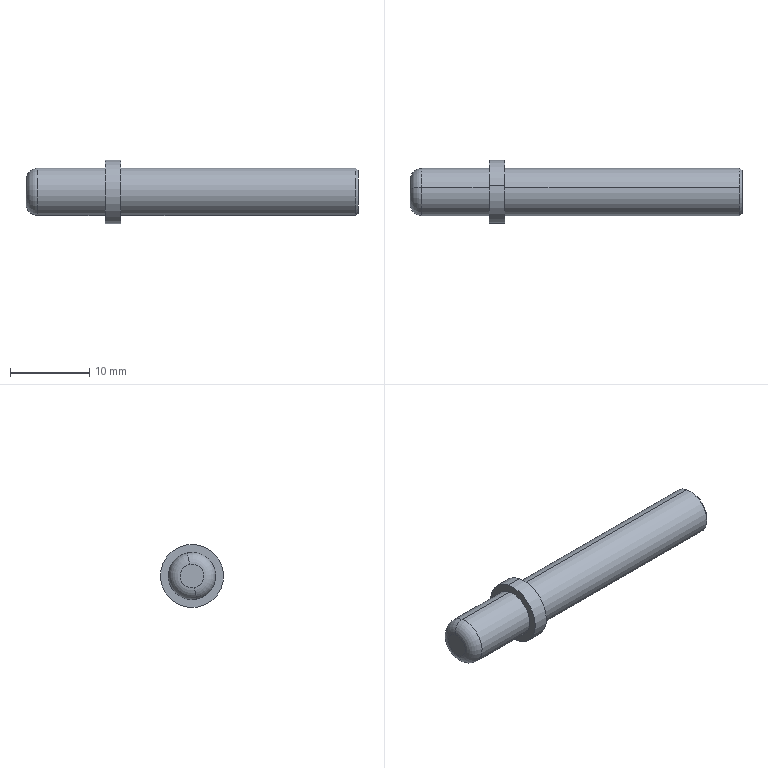Component | SolidWorks | STB-08-000-3-1_STB-08-025-1 | 1 solid | 14 faces | box 42 x 8 x 8 mm | volume 1223 mm3 | cylinder 6 | plane 4 | cone 2 | torus 2 | commonest cylinder face diameters 6 x4 8 x2
build123d program:
from build123d import *

# Parameters (mm, degrees)
SKETCH1_R          = 4
EXTRUDE1_DEPTH     = 42
SKETCH2_OUTSIDE_W  = 18.7
SKETCH2_OUTSIDE_H  = 18.7
SKETCH2_OUTSIDE_R  = 3
CUT_EXTRUDE1_DEPTH = 10
SKETCH3_OUTSIDE_W  = 18.7
SKETCH3_OUTSIDE_H  = 18.7
SKETCH3_OUTSIDE_R  = 3
CUT_EXTRUDE2_DEPTH = 30
FILLET1_R          = 1.5
CHAMFER1_SIZE      = 0.3


with BuildPart() as part:
    # Sketch1 → Extrude1 (new body)
    with BuildSketch(Plane.XY):
        with Locations(Location((0, 0, 0), (0, 0, 180))):
            Circle(SKETCH1_R)
    extrude(amount=EXTRUDE1_DEPTH)

    # Sketch2 outside → Cut-Extrude1 (cut)
    with BuildSketch(Plane.XY.offset(42)):
        Rectangle(SKETCH2_OUTSIDE_W, SKETCH2_OUTSIDE_H)
        Circle(SKETCH2_OUTSIDE_R, mode=Mode.SUBTRACT)
    extrude(amount=-CUT_EXTRUDE1_DEPTH, mode=Mode.SUBTRACT)

    # Sketch3 outside → Cut-Extrude2 (cut)
    with BuildSketch(Plane(origin=(0, 0, 0), x_dir=(-1, 0, 0), z_dir=(0, 0, -1))):
        Rectangle(SKETCH3_OUTSIDE_W, SKETCH3_OUTSIDE_H)
        with Locations(Location((0, 0, 0), (0, 0, 180))):
            Circle(SKETCH3_OUTSIDE_R, mode=Mode.SUBTRACT)
    extrude(amount=-CUT_EXTRUDE2_DEPTH, mode=Mode.SUBTRACT)

    # Fillet1
    fillet1_edges = [part.edges().sort_by_distance(p)[0] for p in [
        (-3, 0, 42),
    ]]
    fillet(fillet1_edges, radius=FILLET1_R)

    # Chamfer1
    chamfer1_edges = [part.edges().sort_by_distance(p)[0] for p in [
        (-3, 0, 0),
    ]]
    chamfer(chamfer1_edges, length=CHAMFER1_SIZE)


solid = part.part

# Placed as in the assembly
solid = solid.moved(Location((-204.904, 437.999, -10), (0, -90, 0)))
STEP:
#1=COLOUR_RGB('',0.7922,0.8196,0.9333);
#2=FILL_AREA_STYLE_COLOUR('',#1);
#3=FILL_AREA_STYLE('',(#2));
#4=SURFACE_STYLE_FILL_AREA(#3);
#5=SURFACE_SIDE_STYLE('',(#4));
#6=SURFACE_STYLE_USAGE(.BOTH.,#5);
#7=PRESENTATION_STYLE_ASSIGNMENT((#6));
#8=CARTESIAN_POINT('',(-8.067,17.223,-0.4979));
#9=VERTEX_POINT('',#8);
#10=CARTESIAN_POINT('',(-8.067,17.265,-0.2895));
#11=VERTEX_POINT('',#10);
#12=CARTESIAN_POINT('',(-8.067,17.244,-0.3937));
#13=DIRECTION('',(1.,-0.,0.));
#14=DIRECTION('',(0.,0.1993,0.9799));
#15=AXIS2_PLACEMENT_3D('',#12,#13,#14);
#16=CIRCLE('',#15,0.1063);
#17=EDGE_CURVE('',#9,#11,#16,.T.);
#18=ORIENTED_EDGE('',*,*,#17,.F.);
#19=CARTESIAN_POINT('',(-8.079,17.221,-0.5094));
#20=VERTEX_POINT('',#19);
#21=CARTESIAN_POINT('',(-8.067,17.223,-0.4979));
#22=DIRECTION('',(-0.7071,-0.1409,-0.6929));
#23=VECTOR('',#22,39.37);
#24=LINE('',#21,#23);
#25=EDGE_CURVE('',#9,#20,#24,.T.);
#26=ORIENTED_EDGE('',*,*,#25,.T.);
#27=CARTESIAN_POINT('',(-8.079,17.268,-0.278));
#28=VERTEX_POINT('',#27);
#29=CARTESIAN_POINT('',(-8.079,17.244,-0.3937));
#30=DIRECTION('',(-1.,0.,-0.));
#31=DIRECTION('',(0.,0.1993,0.9799));
#32=AXIS2_PLACEMENT_3D('',#29,#30,#31);
#33=CIRCLE('',#32,0.1181);
#34=EDGE_CURVE('',#28,#20,#33,.T.);
#35=ORIENTED_EDGE('',*,*,#34,.F.);
#36=CARTESIAN_POINT('',(-8.067,17.265,-0.2895));
#37=DIRECTION('',(-0.7071,0.1409,0.6929));
#38=VECTOR('',#37,39.37);
#39=LINE('',#36,#38);
#40=EDGE_CURVE('',#11,#28,#39,.T.);
#41=ORIENTED_EDGE('',*,*,#40,.F.);
#42=EDGE_LOOP('',(#18,#26,#35,#41));
#43=FACE_OUTER_BOUND('',#42,.T.);
#44=CARTESIAN_POINT('',(-8.067,17.244,-0.3937));
#45=DIRECTION('',(-1.,0.,-0.));
#46=DIRECTION('',(0.,0.1993,0.9799));
#47=AXIS2_PLACEMENT_3D('',#44,#45,#46);
#48=CONICAL_SURFACE('',#47,0.1063,0.7854);
#49=ADVANCED_FACE('',(#43),#48,.T.);
#50=CARTESIAN_POINT('',(-9.662,17.221,-0.5094));
#51=VERTEX_POINT('',#50);
#52=CARTESIAN_POINT('',(-9.662,17.268,-0.278));
#53=VERTEX_POINT('',#52);
#54=CARTESIAN_POINT('',(-9.662,17.244,-0.3937));
#55=DIRECTION('',(1.,-0.,0.));
#56=DIRECTION('',(0.,0.1993,0.9799));
#57=AXIS2_PLACEMENT_3D('',#54,#55,#56);
#58=CIRCLE('',#57,0.1181);
#59=EDGE_CURVE('',#51,#53,#58,.T.);
#60=ORIENTED_EDGE('',*,*,#59,.F.);
#61=CARTESIAN_POINT('',(-9.721,17.232,-0.4516));
#62=VERTEX_POINT('',#61);
#63=CARTESIAN_POINT('',(-9.662,17.232,-0.4516));
#64=DIRECTION('',(0.,0.9799,-0.1993));
#65=DIRECTION('',(0.,0.1993,0.9799));
#66=AXIS2_PLACEMENT_3D('',#63,#64,#65);
#67=CIRCLE('',#66,0.05906);
#68=EDGE_CURVE('',#51,#62,#67,.T.);
#69=ORIENTED_EDGE('',*,*,#68,.T.);
#70=CARTESIAN_POINT('',(-9.721,17.256,-0.3358));
#71=VERTEX_POINT('',#70);
#72=CARTESIAN_POINT('',(-9.721,17.244,-0.3937));
#73=DIRECTION('',(-1.,0.,-0.));
#74=DIRECTION('',(0.,0.1993,0.9799));
#75=AXIS2_PLACEMENT_3D('',#72,#73,#74);
#76=CIRCLE('',#75,0.05906);
#77=EDGE_CURVE('',#71,#62,#76,.T.);
#78=ORIENTED_EDGE('',*,*,#77,.F.);
#79=CARTESIAN_POINT('',(-9.662,17.256,-0.3358));
#80=DIRECTION('',(-0.,-0.9799,0.1993));
#81=DIRECTION('',(0.,-0.1993,-0.9799));
#82=AXIS2_PLACEMENT_3D('',#79,#80,#81);
#83=CIRCLE('',#82,0.05906);
#84=EDGE_CURVE('',#53,#71,#83,.T.);
#85=ORIENTED_EDGE('',*,*,#84,.F.);
#86=EDGE_LOOP('',(#60,#69,#78,#85));
#87=FACE_OUTER_BOUND('',#86,.T.);
#88=CARTESIAN_POINT('',(-9.662,17.244,-0.3937));
#89=DIRECTION('',(-1.,0.,-0.));
#90=DIRECTION('',(0.,0.1993,0.9799));
#91=AXIS2_PLACEMENT_3D('',#88,#89,#90);
#92=TOROIDAL_SURFACE('',#91,0.05906,0.05906);
#93=ADVANCED_FACE('',(#87),#92,.T.);
#94=CARTESIAN_POINT('',(-9.248,17.221,-0.5094));
#95=VERTEX_POINT('',#94);
#96=CARTESIAN_POINT('',(-9.248,17.268,-0.278));
#97=VERTEX_POINT('',#96);
#98=CARTESIAN_POINT('',(-9.248,17.244,-0.3937));
#99=DIRECTION('',(1.,-0.,0.));
#100=DIRECTION('',(0.,-0.1993,-0.9799));
#101=AXIS2_PLACEMENT_3D('',#98,#99,#100);
#102=CIRCLE('',#101,0.1181);
#103=EDGE_CURVE('',#95,#97,#102,.T.);
#104=ORIENTED_EDGE('',*,*,#103,.T.);
#105=CARTESIAN_POINT('',(-9.248,17.268,-0.278));
#106=DIRECTION('',(1.,-0.,0.));
#107=VECTOR('',#106,39.37);
#108=LINE('',#105,#107);
#109=EDGE_CURVE('',#97,#28,#108,.T.);
#110=ORIENTED_EDGE('',*,*,#109,.T.);
#111=ORIENTED_EDGE('',*,*,#34,.T.);
#112=CARTESIAN_POINT('',(-9.248,17.221,-0.5094));
#113=DIRECTION('',(1.,-0.,0.));
#114=VECTOR('',#113,39.37);
#115=LINE('',#112,#114);
#116=EDGE_CURVE('',#95,#20,#115,.T.);
#117=ORIENTED_EDGE('',*,*,#116,.F.);
#118=EDGE_LOOP('',(#104,#110,#111,#117));
#119=FACE_OUTER_BOUND('',#118,.T.);
#120=CARTESIAN_POINT('',(-9.248,17.244,-0.3937));
#121=DIRECTION('',(1.,-0.,0.));
#122=DIRECTION('',(0.,-0.1993,-0.9799));
#123=AXIS2_PLACEMENT_3D('',#120,#121,#122);
#124=CYLINDRICAL_SURFACE('',#123,0.1181);
#125=ADVANCED_FACE('',(#119),#124,.T.);
#126=CARTESIAN_POINT('',(-9.327,17.268,-0.278));
#127=VERTEX_POINT('',#126);
#128=CARTESIAN_POINT('',(-9.327,17.221,-0.5094));
#129=VERTEX_POINT('',#128);
#130=CARTESIAN_POINT('',(-9.327,17.244,-0.3937));
#131=DIRECTION('',(-1.,0.,-0.));
#132=DIRECTION('',(0.,0.1993,0.9799));
#133=AXIS2_PLACEMENT_3D('',#130,#131,#132);
#134=CIRCLE('',#133,0.1181);
#135=EDGE_CURVE('',#127,#129,#134,.T.);
#136=ORIENTED_EDGE('',*,*,#135,.T.);
#137=CARTESIAN_POINT('',(-9.327,17.221,-0.5094));
#138=DIRECTION('',(-1.,0.,-0.));
#139=VECTOR('',#138,39.37);
#140=LINE('',#137,#139);
#141=EDGE_CURVE('',#129,#51,#140,.T.);
#142=ORIENTED_EDGE('',*,*,#141,.T.);
#143=ORIENTED_EDGE('',*,*,#59,.T.);
#144=CARTESIAN_POINT('',(-9.327,17.268,-0.278));
#145=DIRECTION('',(-1.,0.,-0.));
#146=VECTOR('',#145,39.37);
#147=LINE('',#144,#146);
#148=EDGE_CURVE('',#127,#53,#147,.T.);
#149=ORIENTED_EDGE('',*,*,#148,.F.);
#150=EDGE_LOOP('',(#136,#142,#143,#149));
#151=FACE_OUTER_BOUND('',#150,.T.);
#152=CARTESIAN_POINT('',(-9.327,17.244,-0.3937));
#153=DIRECTION('',(-1.,0.,-0.));
#154=DIRECTION('',(0.,0.1993,0.9799));
#155=AXIS2_PLACEMENT_3D('',#152,#153,#154);
#156=CYLINDRICAL_SURFACE('',#155,0.1181);
#157=ADVANCED_FACE('',(#151),#156,.T.);
#158=CARTESIAN_POINT('',(-9.327,17.275,-0.2394));
#159=VERTEX_POINT('',#158);
#160=CARTESIAN_POINT('',(-9.327,17.213,-0.548));
#161=VERTEX_POINT('',#160);
#162=CARTESIAN_POINT('',(-9.327,17.244,-0.3937));
#163=DIRECTION('',(-1.,0.,-0.));
#164=DIRECTION('',(0.,0.1993,0.9799));
#165=AXIS2_PLACEMENT_3D('',#162,#163,#164);
#166=CIRCLE('',#165,0.1575);
#167=EDGE_CURVE('',#159,#161,#166,.T.);
#168=ORIENTED_EDGE('',*,*,#167,.F.);
#169=CARTESIAN_POINT('',(-9.248,17.275,-0.2394));
#170=VERTEX_POINT('',#169);
#171=CARTESIAN_POINT('',(-9.721,17.275,-0.2394));
#172=DIRECTION('',(1.,-0.,0.));
#173=VECTOR('',#172,39.37);
#174=LINE('',#171,#173);
#175=EDGE_CURVE('',#159,#170,#174,.T.);
#176=ORIENTED_EDGE('',*,*,#175,.T.);
#177=CARTESIAN_POINT('',(-9.248,17.213,-0.548));
#178=VERTEX_POINT('',#177);
#179=CARTESIAN_POINT('',(-9.248,17.244,-0.3937));
#180=DIRECTION('',(1.,-0.,0.));
#181=DIRECTION('',(0.,-0.1993,-0.9799));
#182=AXIS2_PLACEMENT_3D('',#179,#180,#181);
#183=CIRCLE('',#182,0.1575);
#184=EDGE_CURVE('',#178,#170,#183,.T.);
#185=ORIENTED_EDGE('',*,*,#184,.F.);
#186=CARTESIAN_POINT('',(-9.721,17.213,-0.548));
#187=DIRECTION('',(1.,-0.,0.));
#188=VECTOR('',#187,39.37);
#189=LINE('',#186,#188);
#190=EDGE_CURVE('',#161,#178,#189,.T.);
#191=ORIENTED_EDGE('',*,*,#190,.F.);
#192=EDGE_LOOP('',(#168,#176,#185,#191));
#193=FACE_OUTER_BOUND('',#192,.T.);
#194=CARTESIAN_POINT('',(-9.721,17.244,-0.3937));
#195=DIRECTION('',(1.,-0.,0.));
#196=DIRECTION('',(0.,-0.1993,-0.9799));
#197=AXIS2_PLACEMENT_3D('',#194,#195,#196);
#198=CYLINDRICAL_SURFACE('',#197,0.1575);
#199=ADVANCED_FACE('',(#193),#198,.T.);
#200=ORIENTED_EDGE('',*,*,#175,.F.);
#201=CARTESIAN_POINT('',(-9.327,17.244,-0.3937));
#202=DIRECTION('',(-1.,0.,-0.));
#203=DIRECTION('',(0.,0.1993,0.9799));
#204=AXIS2_PLACEMENT_3D('',#201,#202,#203);
#205=CIRCLE('',#204,0.1575);
#206=EDGE_CURVE('',#161,#159,#205,.T.);
#207=ORIENTED_EDGE('',*,*,#206,.F.);
#208=ORIENTED_EDGE('',*,*,#190,.T.);
#209=CARTESIAN_POINT('',(-9.248,17.244,-0.3937));
#210=DIRECTION('',(1.,-0.,0.));
#211=DIRECTION('',(0.,-0.1993,-0.9799));
#212=AXIS2_PLACEMENT_3D('',#209,#210,#211);
#213=CIRCLE('',#212,0.1575);
#214=EDGE_CURVE('',#170,#178,#213,.T.);
#215=ORIENTED_EDGE('',*,*,#214,.F.);
#216=EDGE_LOOP('',(#200,#207,#208,#215));
#217=FACE_OUTER_BOUND('',#216,.T.);
#218=CARTESIAN_POINT('',(-9.721,17.244,-0.3937));
#219=DIRECTION('',(1.,-0.,0.));
#220=DIRECTION('',(0.,-0.1993,-0.9799));
#221=AXIS2_PLACEMENT_3D('',#218,#219,#220);
#222=CYLINDRICAL_SURFACE('',#221,0.1575);
#223=ADVANCED_FACE('',(#217),#222,.T.);
#224=ORIENTED_EDGE('',*,*,#135,.F.);
#225=CARTESIAN_POINT('',(-9.327,17.244,-0.3937));
#226=DIRECTION('',(-1.,0.,-0.));
#227=DIRECTION('',(0.,0.1993,0.9799));
#228=AXIS2_PLACEMENT_3D('',#225,#226,#227);
#229=CIRCLE('',#228,0.1181);
#230=EDGE_CURVE('',#129,#127,#229,.T.);
#231=ORIENTED_EDGE('',*,*,#230,.F.);
#232=EDGE_LOOP('',(#224,#231));
#233=FACE_BOUND('',#232,.T.);
#234=ORIENTED_EDGE('',*,*,#206,.T.);
#235=ORIENTED_EDGE('',*,*,#167,.T.);
#236=EDGE_LOOP('',(#234,#235));
#237=FACE_OUTER_BOUND('',#236,.T.);
#238=CARTESIAN_POINT('',(-9.327,17.244,-0.3937));
#239=DIRECTION('',(-1.,0.,-0.));
#240=DIRECTION('',(-0.,0.1993,0.9799));
#241=AXIS2_PLACEMENT_3D('',#238,#239,#240);
#242=PLANE('',#241);
#243=ADVANCED_FACE('',(#233,#237),#242,.T.);
#244=ORIENTED_EDGE('',*,*,#141,.F.);
#245=ORIENTED_EDGE('',*,*,#230,.T.);
#246=ORIENTED_EDGE('',*,*,#148,.T.);
#247=CARTESIAN_POINT('',(-9.662,17.244,-0.3937));
#248=DIRECTION('',(1.,-0.,0.));
#249=DIRECTION('',(0.,0.1993,0.9799));
#250=AXIS2_PLACEMENT_3D('',#247,#248,#249);
#251=CIRCLE('',#250,0.1181);
#252=EDGE_CURVE('',#53,#51,#251,.T.);
#253=ORIENTED_EDGE('',*,*,#252,.T.);
#254=EDGE_LOOP('',(#244,#245,#246,#253));
#255=FACE_OUTER_BOUND('',#254,.T.);
#256=CARTESIAN_POINT('',(-9.327,17.244,-0.3937));
#257=DIRECTION('',(-1.,0.,-0.));
#258=DIRECTION('',(0.,0.1993,0.9799));
#259=AXIS2_PLACEMENT_3D('',#256,#257,#258);
#260=CYLINDRICAL_SURFACE('',#259,0.1181);
#261=ADVANCED_FACE('',(#255),#260,.T.);
#262=ORIENTED_EDGE('',*,*,#77,.T.);
#263=CARTESIAN_POINT('',(-9.721,17.244,-0.3937));
#264=DIRECTION('',(-1.,0.,-0.));
#265=DIRECTION('',(0.,0.1993,0.9799));
#266=AXIS2_PLACEMENT_3D('',#263,#264,#265);
#267=CIRCLE('',#266,0.05906);
#268=EDGE_CURVE('',#62,#71,#267,.T.);
#269=ORIENTED_EDGE('',*,*,#268,.T.);
#270=EDGE_LOOP('',(#262,#269));
#271=FACE_OUTER_BOUND('',#270,.T.);
#272=CARTESIAN_POINT('',(-9.721,17.244,-0.3937));
#273=DIRECTION('',(-1.,0.,-0.));
#274=DIRECTION('',(-0.,0.1993,0.9799));
#275=AXIS2_PLACEMENT_3D('',#272,#273,#274);
#276=PLANE('',#275);
#277=ADVANCED_FACE('',(#271),#276,.T.);
#278=ORIENTED_EDGE('',*,*,#103,.F.);
#279=CARTESIAN_POINT('',(-9.248,17.244,-0.3937));
#280=DIRECTION('',(1.,-0.,0.));
#281=DIRECTION('',(0.,-0.1993,-0.9799));
#282=AXIS2_PLACEMENT_3D('',#279,#280,#281);
#283=CIRCLE('',#282,0.1181);
#284=EDGE_CURVE('',#97,#95,#283,.T.);
#285=ORIENTED_EDGE('',*,*,#284,.F.);
#286=EDGE_LOOP('',(#278,#285));
#287=FACE_BOUND('',#286,.T.);
#288=ORIENTED_EDGE('',*,*,#184,.T.);
#289=ORIENTED_EDGE('',*,*,#214,.T.);
#290=EDGE_LOOP('',(#288,#289));
#291=FACE_OUTER_BOUND('',#290,.T.);
#292=CARTESIAN_POINT('',(-9.248,17.244,-0.3937));
#293=DIRECTION('',(1.,-0.,0.));
#294=DIRECTION('',(0.,-0.1993,-0.9799));
#295=AXIS2_PLACEMENT_3D('',#292,#293,#294);
#296=PLANE('',#295);
#297=ADVANCED_FACE('',(#287,#291),#296,.T.);
#298=ORIENTED_EDGE('',*,*,#109,.F.);
#299=ORIENTED_EDGE('',*,*,#284,.T.);
#300=ORIENTED_EDGE('',*,*,#116,.T.);
#301=CARTESIAN_POINT('',(-8.079,17.244,-0.3937));
#302=DIRECTION('',(-1.,0.,-0.));
#303=DIRECTION('',(0.,0.1993,0.9799));
#304=AXIS2_PLACEMENT_3D('',#301,#302,#303);
#305=CIRCLE('',#304,0.1181);
#306=EDGE_CURVE('',#20,#28,#305,.T.);
#307=ORIENTED_EDGE('',*,*,#306,.T.);
#308=EDGE_LOOP('',(#298,#299,#300,#307));
#309=FACE_OUTER_BOUND('',#308,.T.);
#310=CARTESIAN_POINT('',(-9.248,17.244,-0.3937));
#311=DIRECTION('',(1.,-0.,0.));
#312=DIRECTION('',(0.,-0.1993,-0.9799));
#313=AXIS2_PLACEMENT_3D('',#310,#311,#312);
#314=CYLINDRICAL_SURFACE('',#313,0.1181);
#315=ADVANCED_FACE('',(#309),#314,.T.);
#316=CARTESIAN_POINT('',(-8.067,17.244,-0.3937));
#317=DIRECTION('',(1.,-0.,0.));
#318=DIRECTION('',(0.,0.1993,0.9799));
#319=AXIS2_PLACEMENT_3D('',#316,#317,#318);
#320=CIRCLE('',#319,0.1063);
#321=EDGE_CURVE('',#11,#9,#320,.T.);
#322=ORIENTED_EDGE('',*,*,#321,.T.);
#323=ORIENTED_EDGE('',*,*,#17,.T.);
#324=EDGE_LOOP('',(#322,#323));
#325=FACE_OUTER_BOUND('',#324,.T.);
#326=CARTESIAN_POINT('',(-8.067,17.244,-0.3937));
#327=DIRECTION('',(-1.,0.,-0.));
#328=DIRECTION('',(-0.,0.1993,0.9799));
#329=AXIS2_PLACEMENT_3D('',#326,#327,#328);
#330=PLANE('',#329);
#331=ADVANCED_FACE('',(#325),#330,.F.);
#332=ORIENTED_EDGE('',*,*,#68,.F.);
#333=ORIENTED_EDGE('',*,*,#252,.F.);
#334=ORIENTED_EDGE('',*,*,#84,.T.);
#335=ORIENTED_EDGE('',*,*,#268,.F.);
#336=EDGE_LOOP('',(#332,#333,#334,#335));
#337=FACE_OUTER_BOUND('',#336,.T.);
#338=CARTESIAN_POINT('',(-9.662,17.244,-0.3937));
#339=DIRECTION('',(-1.,0.,-0.));
#340=DIRECTION('',(0.,0.1993,0.9799));
#341=AXIS2_PLACEMENT_3D('',#338,#339,#340);
#342=TOROIDAL_SURFACE('',#341,0.05906,0.05906);
#343=ADVANCED_FACE('',(#337),#342,.T.);
#344=ORIENTED_EDGE('',*,*,#25,.F.);
#345=ORIENTED_EDGE('',*,*,#321,.F.);
#346=ORIENTED_EDGE('',*,*,#40,.T.);
#347=ORIENTED_EDGE('',*,*,#306,.F.);
#348=EDGE_LOOP('',(#344,#345,#346,#347));
#349=FACE_OUTER_BOUND('',#348,.T.);
#350=CARTESIAN_POINT('',(-8.067,17.244,-0.3937));
#351=DIRECTION('',(-1.,0.,-0.));
#352=DIRECTION('',(0.,0.1993,0.9799));
#353=AXIS2_PLACEMENT_3D('',#350,#351,#352);
#354=CONICAL_SURFACE('',#353,0.1063,0.7854);
#355=ADVANCED_FACE('',(#349),#354,.T.);
#356=CLOSED_SHELL('',(#49,#93,#125,#157,#199,#223,#243,#261,#277,#297,#315,#331,#343,#355));
#357=MANIFOLD_SOLID_BREP('',#356);
#358=STYLED_ITEM('',(#7),#357);
#359=(LENGTH_UNIT()NAMED_UNIT(*)SI_UNIT($,.METRE.));
#360=LENGTH_MEASURE_WITH_UNIT(LENGTH_MEASURE(0.0254),#359);
#361=DIMENSIONAL_EXPONENTS(1.,0.,0.,0.,0.,0.,0.);
#362=(CONVERSION_BASED_UNIT('',#360)LENGTH_UNIT()NAMED_UNIT(#361));
#363=UNCERTAINTY_MEASURE_WITH_UNIT(LENGTH_MEASURE(0.00001),#362,'','');
#364=(NAMED_UNIT(*)PLANE_ANGLE_UNIT()SI_UNIT($,.RADIAN.));
#365=(NAMED_UNIT(*)SI_UNIT($,.STERADIAN.)SOLID_ANGLE_UNIT());
#366=(GEOMETRIC_REPRESENTATION_CONTEXT(3)GLOBAL_UNCERTAINTY_ASSIGNED_CONTEXT((#363))GLOBAL_UNIT_ASSIGNED_CONTEXT((#362,#364,#365))REPRESENTATION_CONTEXT('',''));
#367=MECHANICAL_DESIGN_GEOMETRIC_PRESENTATION_REPRESENTATION('',(#358),#366);
#368=CARTESIAN_POINT('',(0.,0.,0.));
#369=DIRECTION('',(0.,0.,1.));
#370=DIRECTION('',(1.,0.,0.));
#371=AXIS2_PLACEMENT_3D('',#368,#369,#370);
#372=(LENGTH_UNIT()NAMED_UNIT(*)SI_UNIT($,.METRE.));
#373=LENGTH_MEASURE_WITH_UNIT(LENGTH_MEASURE(0.0254),#372);
#374=DIMENSIONAL_EXPONENTS(1.,0.,0.,0.,0.,0.,0.);
#375=(CONVERSION_BASED_UNIT('',#373)LENGTH_UNIT()NAMED_UNIT(#374));
#376=UNCERTAINTY_MEASURE_WITH_UNIT(LENGTH_MEASURE(0.00001),#375,'','');
#377=(NAMED_UNIT(*)PLANE_ANGLE_UNIT()SI_UNIT($,.RADIAN.));
#378=(NAMED_UNIT(*)SI_UNIT($,.STERADIAN.)SOLID_ANGLE_UNIT());
#379=(GEOMETRIC_REPRESENTATION_CONTEXT(3)GLOBAL_UNCERTAINTY_ASSIGNED_CONTEXT((#376))GLOBAL_UNIT_ASSIGNED_CONTEXT((#375,#377,#378))REPRESENTATION_CONTEXT('',''));
#380=ADVANCED_BREP_SHAPE_REPRESENTATION('',(#357,#371),#379);
#381=PRESENTATION_LAYER_ASSIGNMENT('','',(#358));